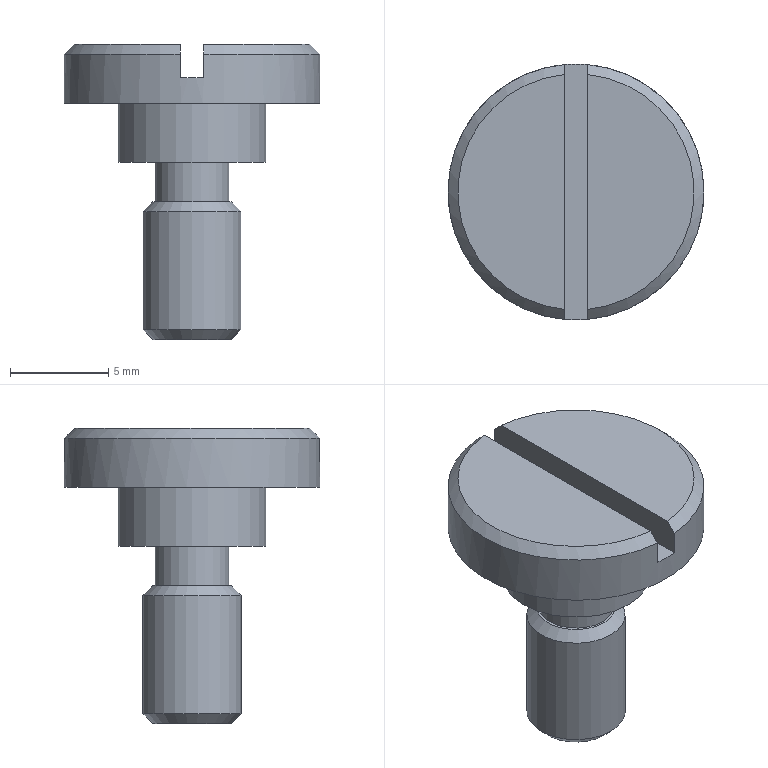Component | NX | DRILL_BUSH_SCREW | 1 solid | 17 faces | volume 655 mm3 | plane 9 | cylinder 4 | cone 4 | commonest cylinder face diameters 5 x1 3.75 x1 7.5 x1 13 x1